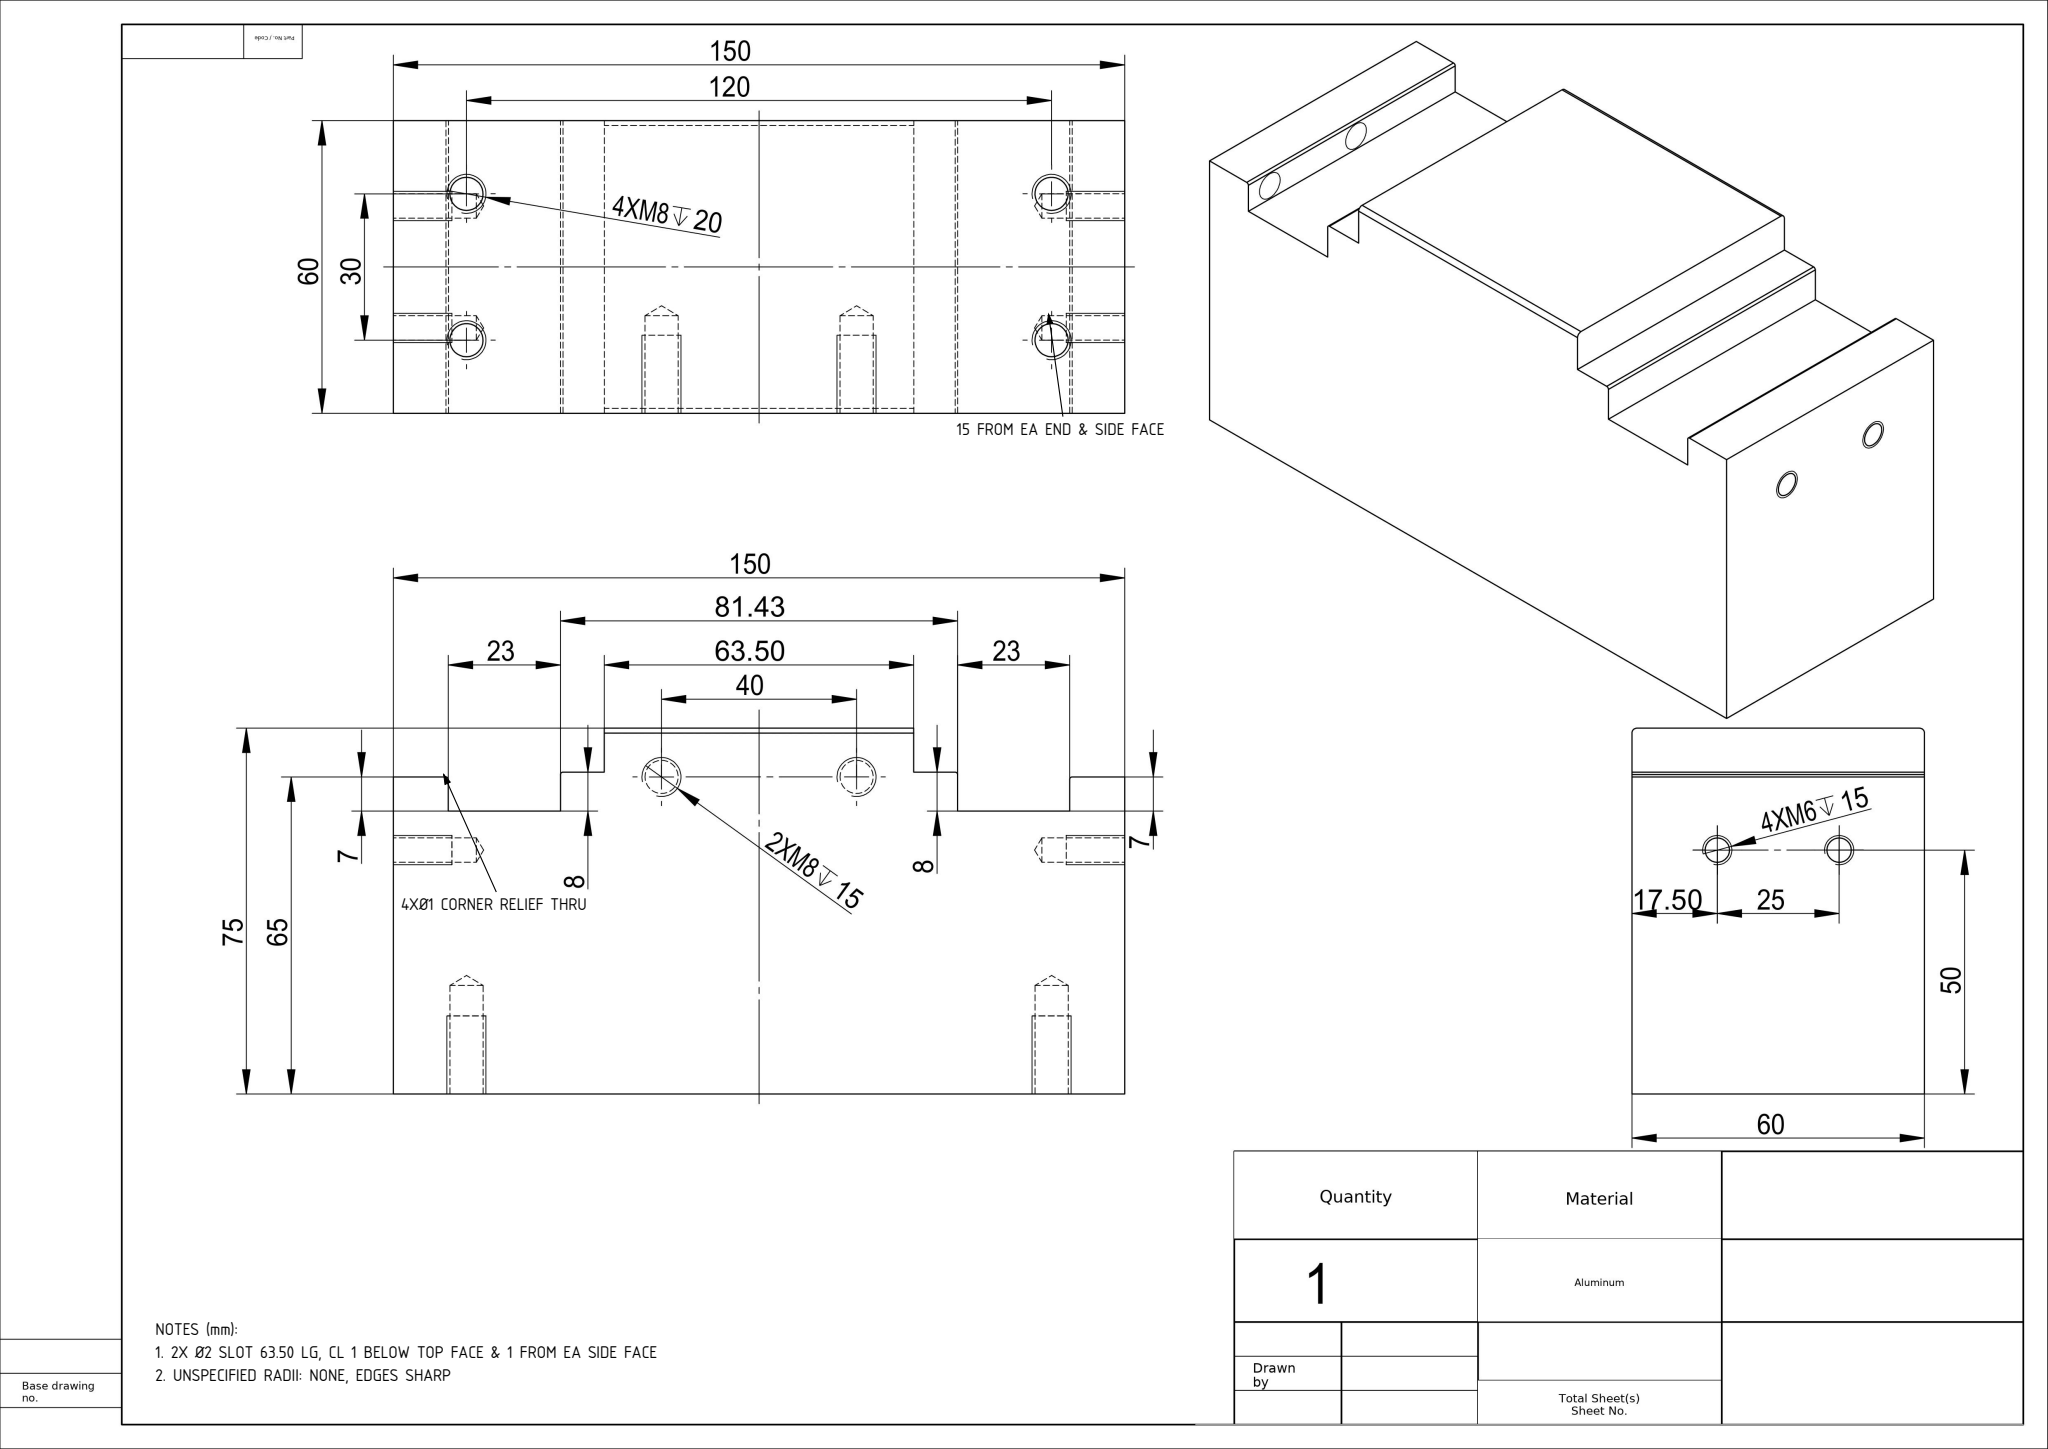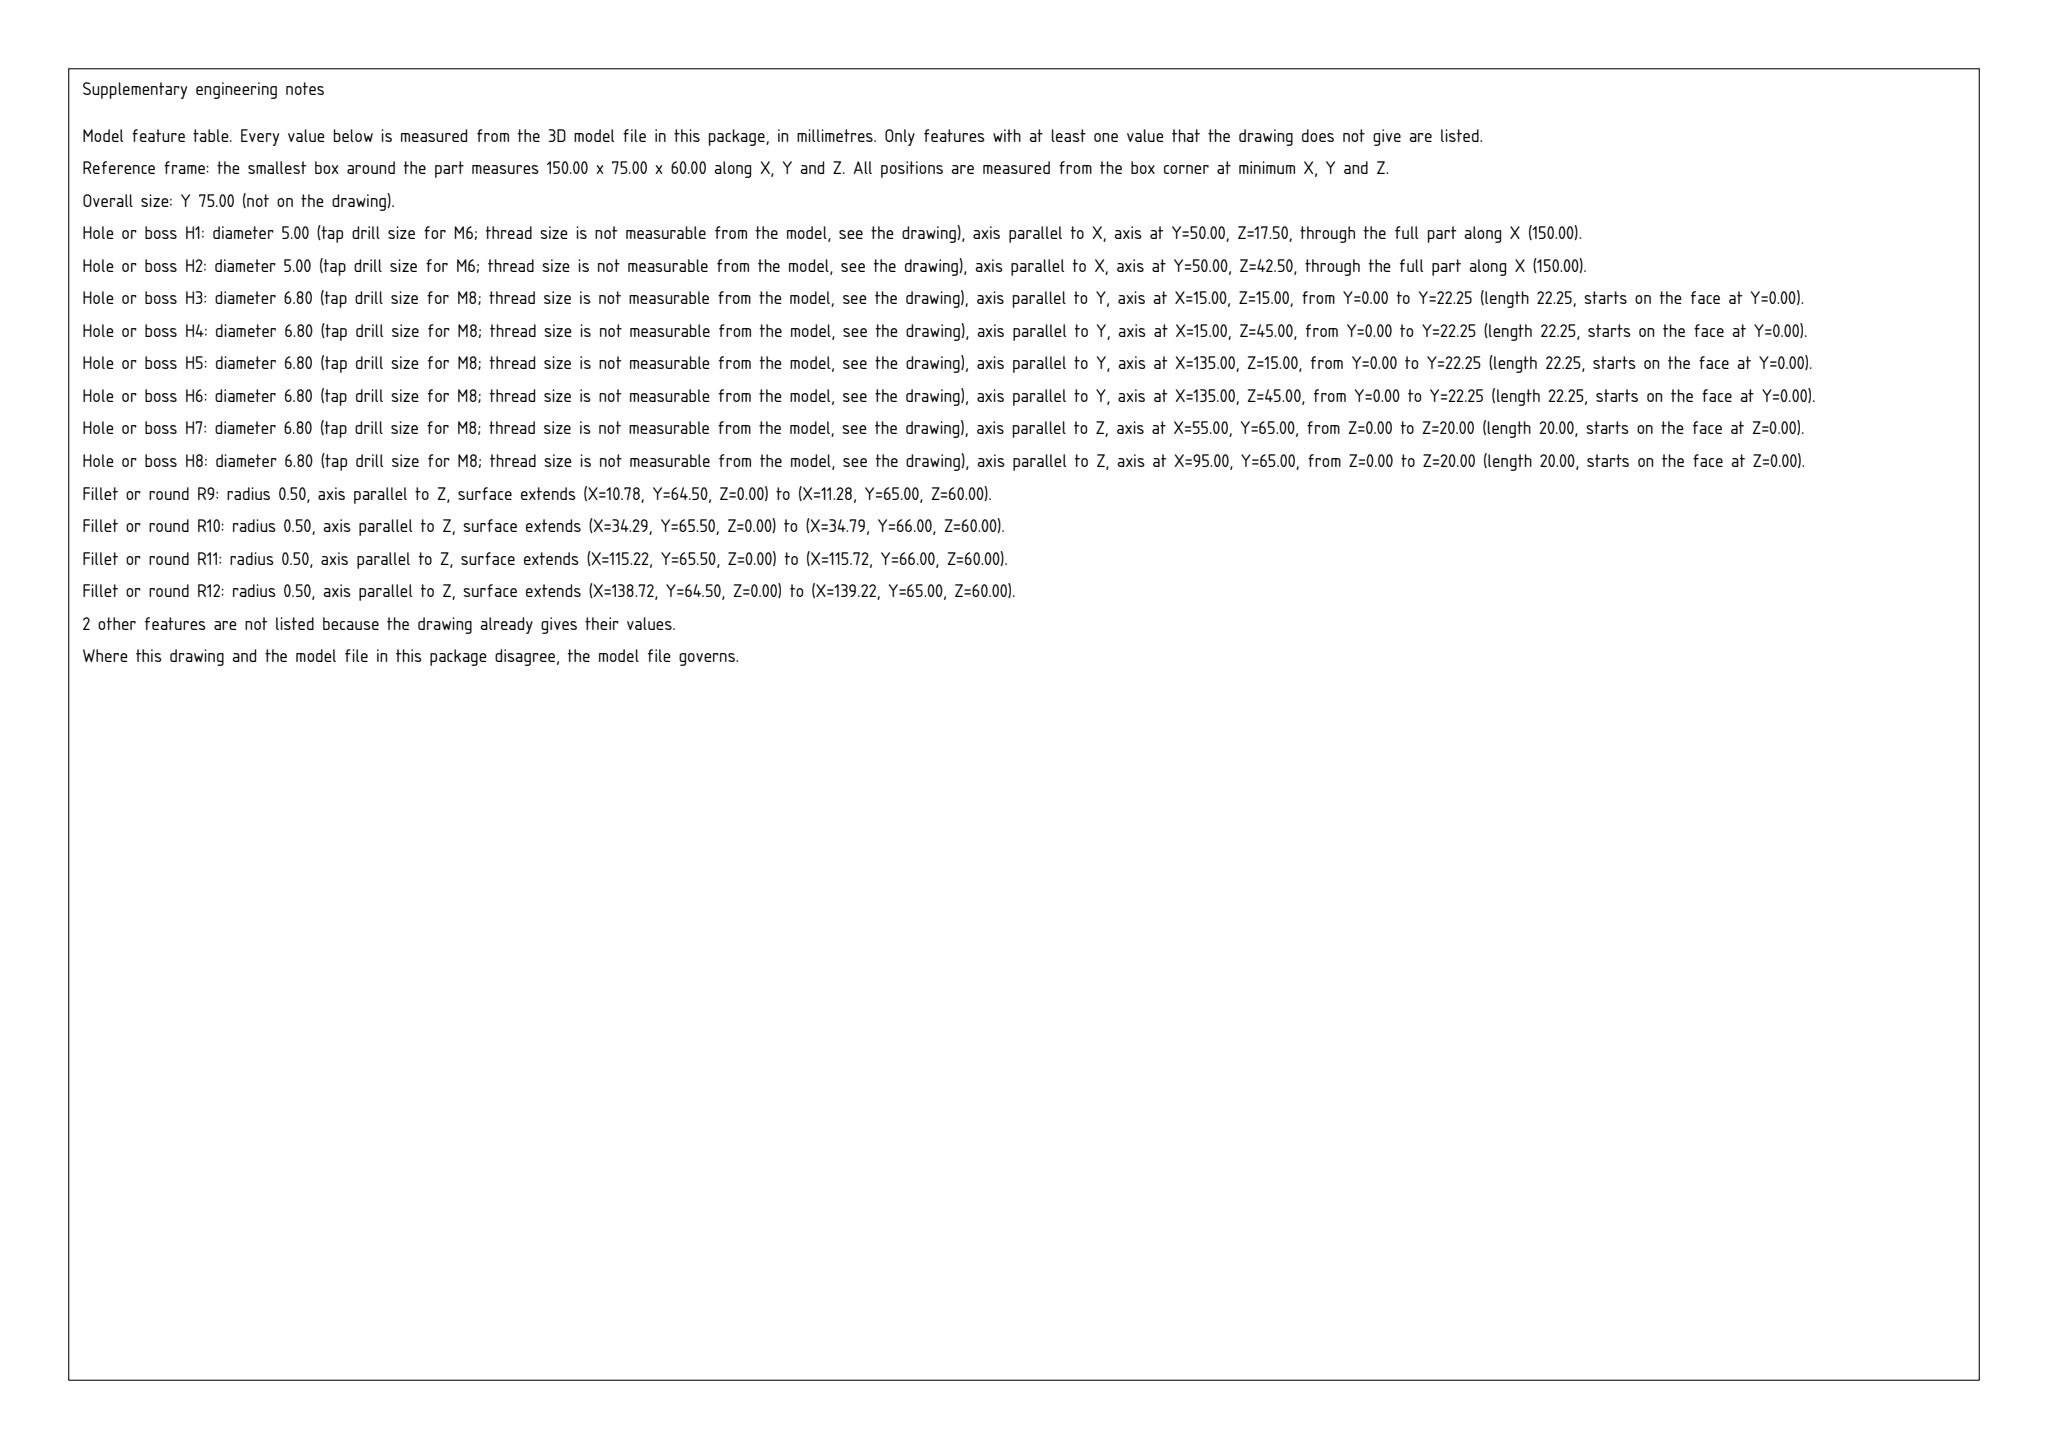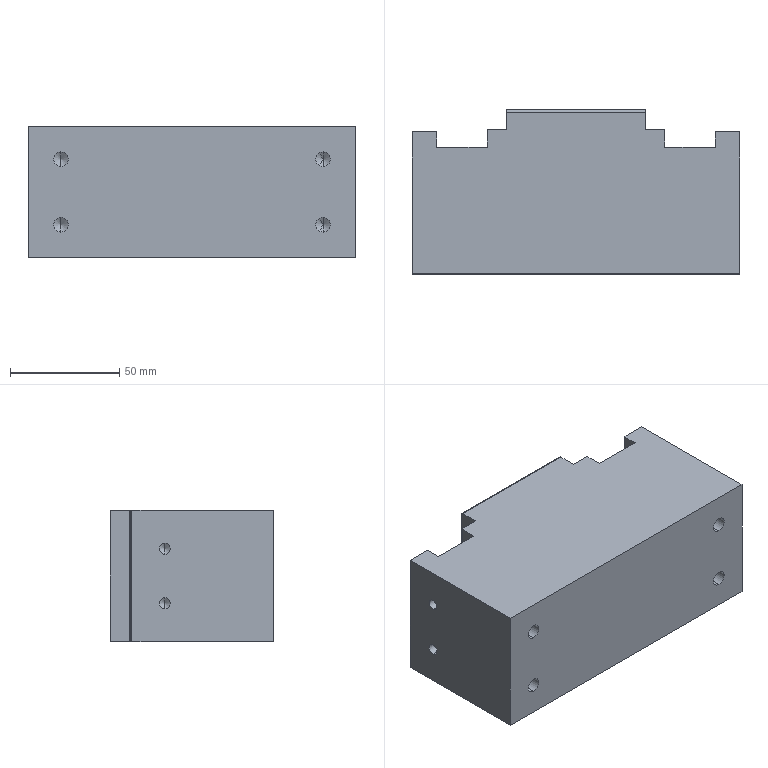Part | SolidWorks | mm | material Aluminum | 1 solid | 64 faces | box 150 x 75 x 60 mm | volume 598589 mm3 | cylinder 26 | cone 20 | plane 18 | commonest cylinder face diameters 6.8 x12 5 x8 1 x4 2 x2
Drawing notes:
2X Ø2 SLOT 63.50 LG, CL 1 BELOW TOP FACE & 1 FROM EA SIDE FACE | from the solid: cylinders [2.0,"x",[null,74.0,1.0],63.49] and [2.0,"x",[null,74.0,59.0],63.49]; bbox Y=75 top face, Z=0/60 side faces; 63.49 length spans x 43.26-106.74, matching 63.50
4XM8 DP 20, CL 15 FROM EA END FACE & 15 FROM EA SIDE FACE | from the solid: cylinders Ø6.8 axis y at x=15/135, z=15/45, length 22.25 with 118 deg point (tap drill for M8 DP 20); bbox 150 x 75 x 60
4X Ø1 CORNER RELIEF THRU 60 AT STEP WALLS, TANGENT TO 65 FACE | from the solid: cylinders dia 1.0 axis z, len 60 at (10.78,64.5),(34.79,65.5),(115.22,65.5),(139.22,64.5); step faces y=65, walls x=11.28/34.29/115.72/138.72
UNSPECIFIED RADII: NONE, EDGES SHARP | from the solid: fillet_radii list empty in STEP data
build123d program:
from build123d import *

# Parameters (mm, degrees)
SKETCH1_W                  = 150
SKETCH1_H                  = 60
BOSS_EXTRUDE1_DEPTH        = 75
SKETCH2_W                  = 22.974
SKETCH2_H                  = 17.004
CUT_EXTRUDE1_DEPTH         = 179.115
SKETCH3_W                  = 11.282
SKETCH3_H                  = 10
CUT_EXTRUDE2_DEPTH         = 179.115
SKETCH4_W                  = 10
SKETCH4_H                  = 9
CUT_EXTRUDE3_DEPTH         = 179.115
SKETCH6_W                  = 60
SKETCH6_H                  = 9
BOSS_EXTRUDE2_DEPTH        = 1
SKETCH7_W                  = 60
SKETCH7_H                  = 17.004
CUT_EXTRUDE5_DEPTH         = 9
M6_TAPPED_HOLE1_AT_2_COUNT = 2
M6_TAPPED_HOLE1_AT_2_PITCH = 25
M8_TAPPED_HOLE1_D          = 6.8
M8_TAPPED_HOLE1_DEPTH      = 20
M8_TAPPED_HOLE1_TIP        = 2.043
M8_TAPPED_HOLE2_D          = 6.8
M8_TAPPED_HOLE2_DEPTH      = 22.25
M8_TAPPED_HOLE2_TIP        = 2.043
FILLET2_R                  = 1
SKETCH18_W                 = 8.974
SKETCH18_H                 = 8.004
BOSS_EXTRUDE3_DEPTH        = 60
SKETCH19_W                 = 60
SKETCH19_H                 = 8.004
CUT_EXTRUDE6_DEPTH         = 0.03
FILLET3_R                  = 0.5
FILLET4_R                  = 0.5


with BuildPart() as part:
    # Sketch1 → Boss-Extrude1 (new body)
    with BuildSketch(Plane(origin=(0, 0, 0), x_dir=(1, 0, 0), z_dir=(0, 1, 0))):
        with Locations((-75, 30)):
            Rectangle(SKETCH1_W, SKETCH1_H)
    extrude(amount=BOSS_EXTRUDE1_DEPTH)

    # Sketch2 → Cut-Extrude1 (cut, through all)
    with BuildSketch(Plane.XY):
        with Locations((-127.231, 66.498)):
            Rectangle(SKETCH2_W, SKETCH2_H)
    cut_extrude1 = extrude(amount=-CUT_EXTRUDE1_DEPTH, mode=Mode.SUBTRACT)

    # Mirror1: Cut-Extrude1 across plane
    add(cut_extrude1.mirror(Plane(origin=(-75, 0, 0), x_dir=(0, 0, 1), z_dir=(1, 0, 0))), mode=Mode.SUBTRACT)

    # Sketch3 → Cut-Extrude2 (cut, through all)
    with BuildSketch(Plane.XY):
        with Locations((-144.359, 70)):
            Rectangle(SKETCH3_W, SKETCH3_H)
        with Locations((-5.641, 70)):
            Rectangle(SKETCH3_W, SKETCH3_H)
    extrude(amount=-CUT_EXTRUDE2_DEPTH, mode=Mode.SUBTRACT)

    # Sketch4 → Cut-Extrude3 (cut, through all)
    with BuildSketch(Plane.XY):
        with Locations((-110.744, 70.5)):
            Rectangle(SKETCH4_W, SKETCH4_H)
    extrude(amount=-CUT_EXTRUDE3_DEPTH, mode=Mode.SUBTRACT)

    # Sketch6 → Boss-Extrude2 (add)
    with BuildSketch(Plane.ZY.offset(105.744)):
        with Locations((-30, 70.5)):
            Rectangle(SKETCH6_W, SKETCH6_H)
    extrude(amount=BOSS_EXTRUDE2_DEPTH)

    # Sketch7 → Cut-Extrude5 (cut)
    with BuildSketch(Plane(origin=(-34.256, 0, 0), x_dir=(0, 0, -1), z_dir=(1, 0, 0))):
        with Locations((30, 66.498)):
            Rectangle(SKETCH7_W, SKETCH7_H)
    extrude(amount=-CUT_EXTRUDE5_DEPTH, mode=Mode.SUBTRACT)

    # Sketch10 → M6 Tapped Hole1 (revolve, cut)
    with BuildSketch(Plane(origin=(-150, 50, -42.5), x_dir=(0, 0, 1), z_dir=(0, 1, 0))):
        Polygon((0, 0), (0, 18.502), (2.5, 17), (2.5, 0), align=None)
    m6_tapped_hole1 = revolve(axis=Axis((-156.35, 50, -42.5), (1, 0, 0)), mode=Mode.SUBTRACT)

    # M6 Tapped Hole1 at 2: M6 Tapped Hole1 ×2
    with Locations(*[(0, 0, i * M6_TAPPED_HOLE1_AT_2_PITCH) for i in range(1, M6_TAPPED_HOLE1_AT_2_COUNT)]):
        add(m6_tapped_hole1, mode=Mode.SUBTRACT)

    # Mirror2: M6 Tapped Hole1 across plane
    add(m6_tapped_hole1.mirror(Plane.ZY.offset(75)), mode=Mode.SUBTRACT)

    # Mirror2 copy 1 sketch → Mirror2 copy 1 (revolve, cut)
    with BuildSketch(Plane(origin=(0, 50, -17.5), x_dir=(0, 0, 1), z_dir=(0, 1, 0))):
        Polygon((0, 0), (0, -18.502), (2.5, -17), (2.5, 0), align=None)
    revolve(axis=Axis((6.35, 50, -17.5), (1, 0, 0)), mode=Mode.SUBTRACT)

    # M8 Tapped Hole1
    with Locations(Plane(origin=(0, 0, -60), x_dir=(-1, 0, 0), z_dir=(0, 0, -1))):
        with Locations((55, 64.996), (95, 64.996)):
            Hole(M8_TAPPED_HOLE1_D / 2, depth=M8_TAPPED_HOLE1_DEPTH)
            with Locations((0, 0, -(M8_TAPPED_HOLE1_DEPTH + M8_TAPPED_HOLE1_TIP / 2))):  # 118° drill point
                Cone(0, M8_TAPPED_HOLE1_D / 2, M8_TAPPED_HOLE1_TIP, mode=Mode.SUBTRACT)

    # M8 Tapped Hole2
    with Locations(Plane(origin=(0, 0, 0), x_dir=(-1, 0, 0), z_dir=(0, -1, 0))):
        with Locations((135, 15), (135, 45), (15, 15), (15, 45)):
            Hole(M8_TAPPED_HOLE2_D / 2, depth=M8_TAPPED_HOLE2_DEPTH)
            with Locations((0, 0, -(M8_TAPPED_HOLE2_DEPTH + M8_TAPPED_HOLE2_TIP / 2))):  # 118° drill point
                Cone(0, M8_TAPPED_HOLE2_D / 2, M8_TAPPED_HOLE2_TIP, mode=Mode.SUBTRACT)

    # Fillet2
    fillet2_edges = [part.edges().sort_by_distance(p)[0] for p in [
        (-75, 75, 0),
        (-75, 75, -60),
    ]]
    fillet(fillet2_edges, radius=FILLET2_R)

    # Sketch18 → Boss-Extrude3 (add)
    with BuildSketch(Plane.XY):
        with Locations((-38.769, 61.998)):
            Rectangle(SKETCH18_W, SKETCH18_H)
    extrude(amount=-BOSS_EXTRUDE3_DEPTH)

    # Sketch19 → Cut-Extrude6 (cut)
    with BuildSketch(Plane.ZY.offset(115.744)):
        with Locations((-30, 61.998)):
            Rectangle(SKETCH19_W, SKETCH19_H)
    extrude(amount=-CUT_EXTRUDE6_DEPTH, mode=Mode.SUBTRACT)

    # Fillet3
    fillet3_edges = [part.edges().sort_by_distance(p)[0] for p in [
        (-115.714, 66, -30),
        (-138.718, 65, -30),
    ]]
    fillet(fillet3_edges, radius=FILLET3_R)

    # Fillet4
    fillet4_edges = [part.edges().sort_by_distance(p)[0] for p in [
        (-34.282, 66, -30),
        (-11.282, 65, -30),
    ]]
    fillet(fillet4_edges, radius=FILLET4_R)


solid = part.part